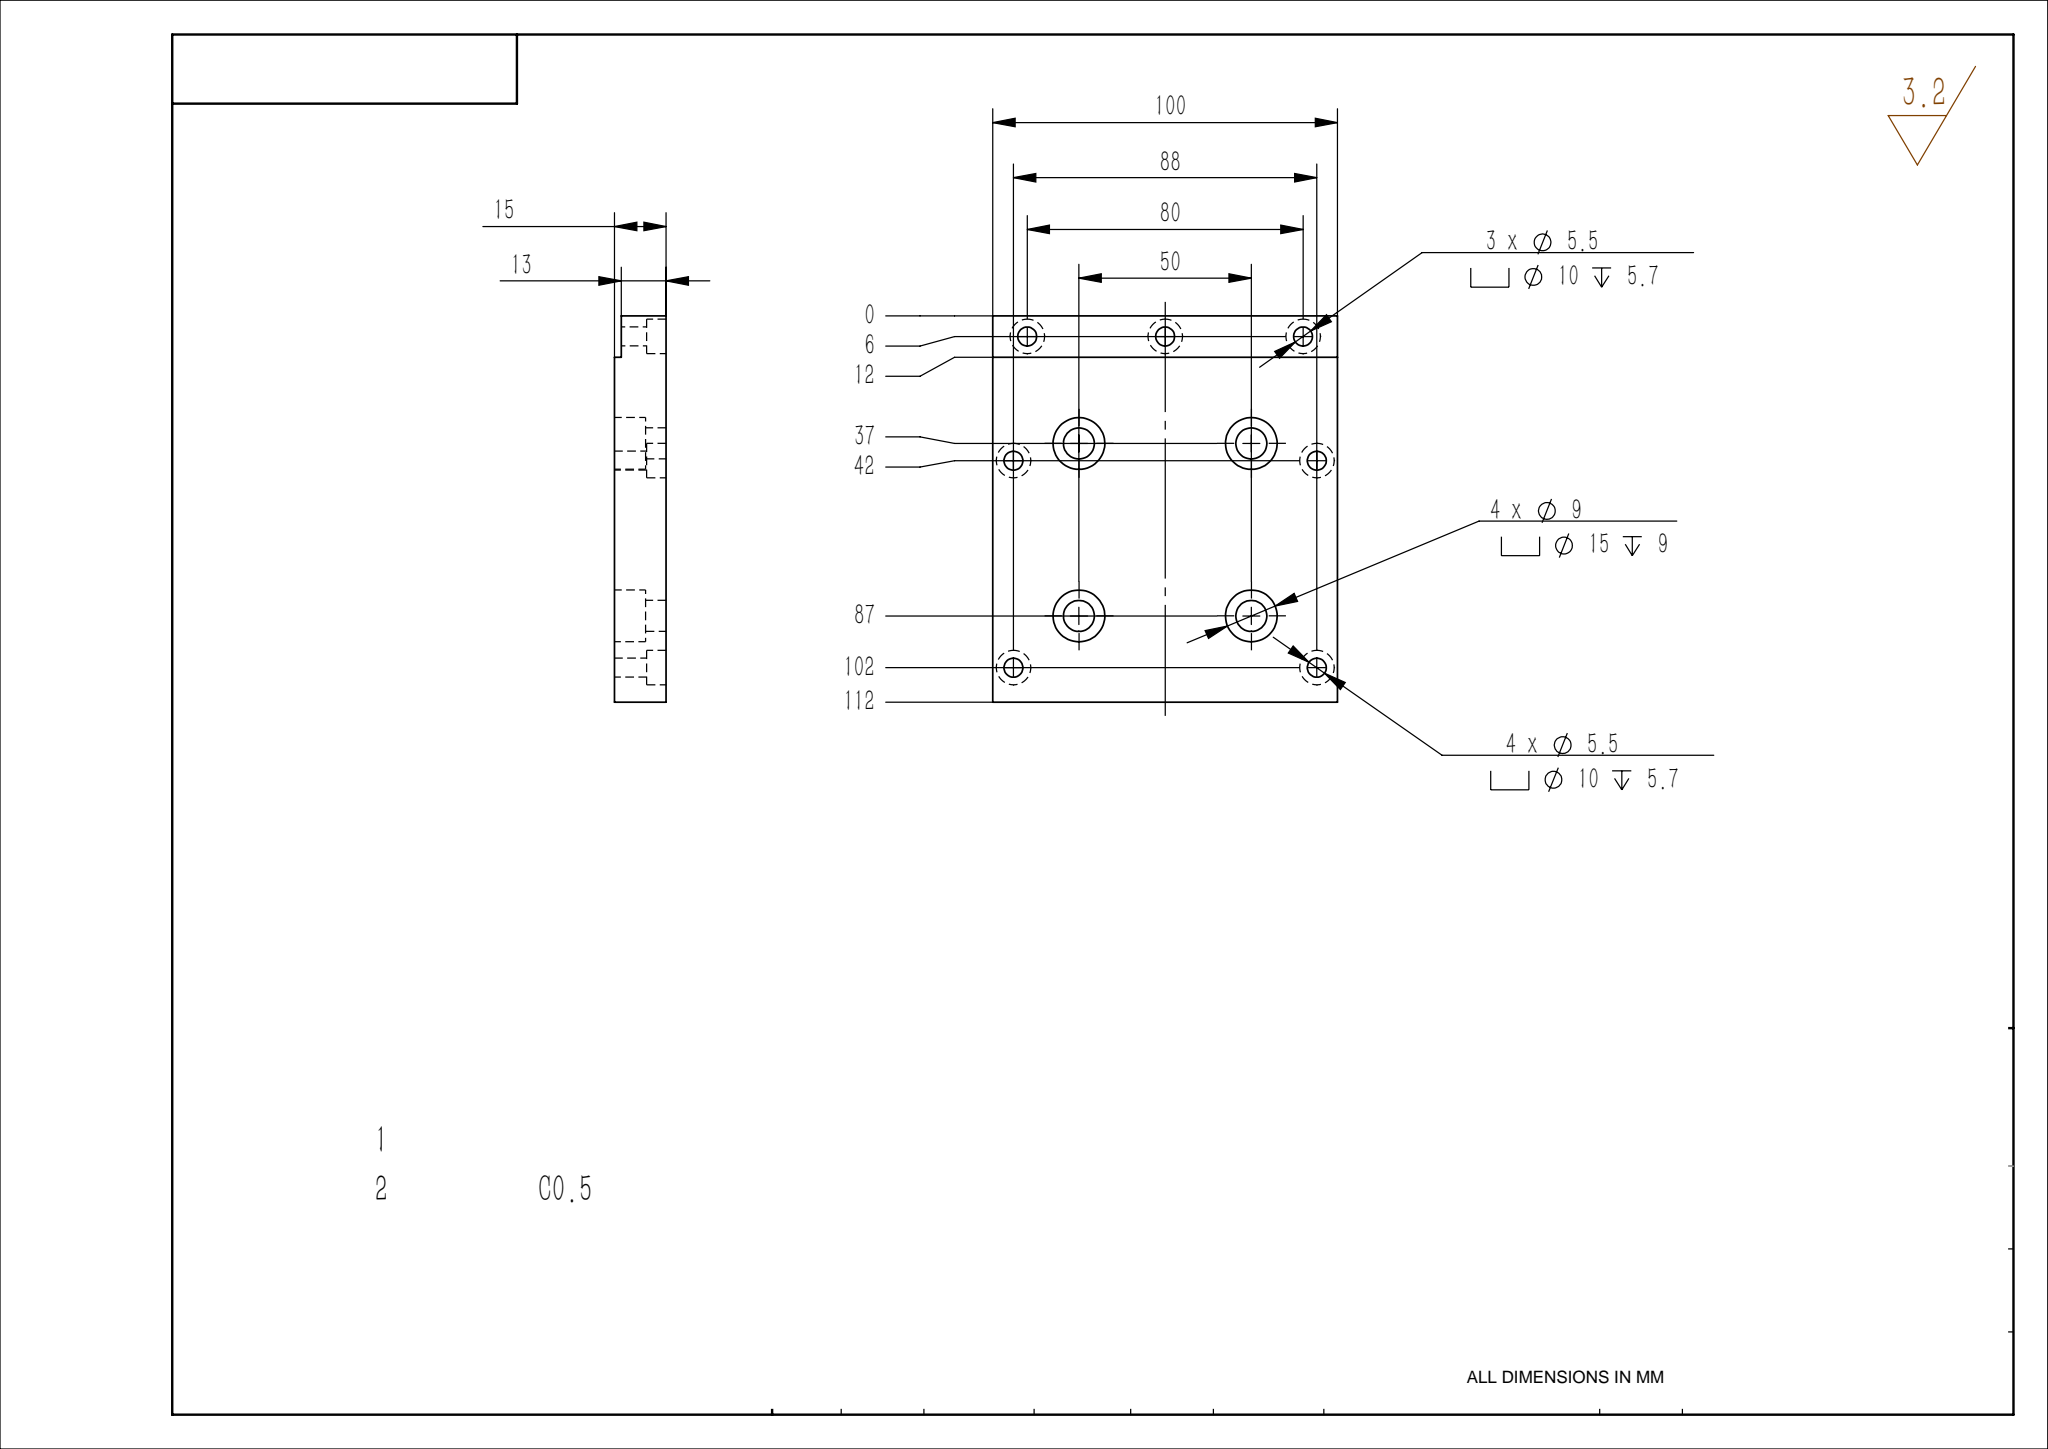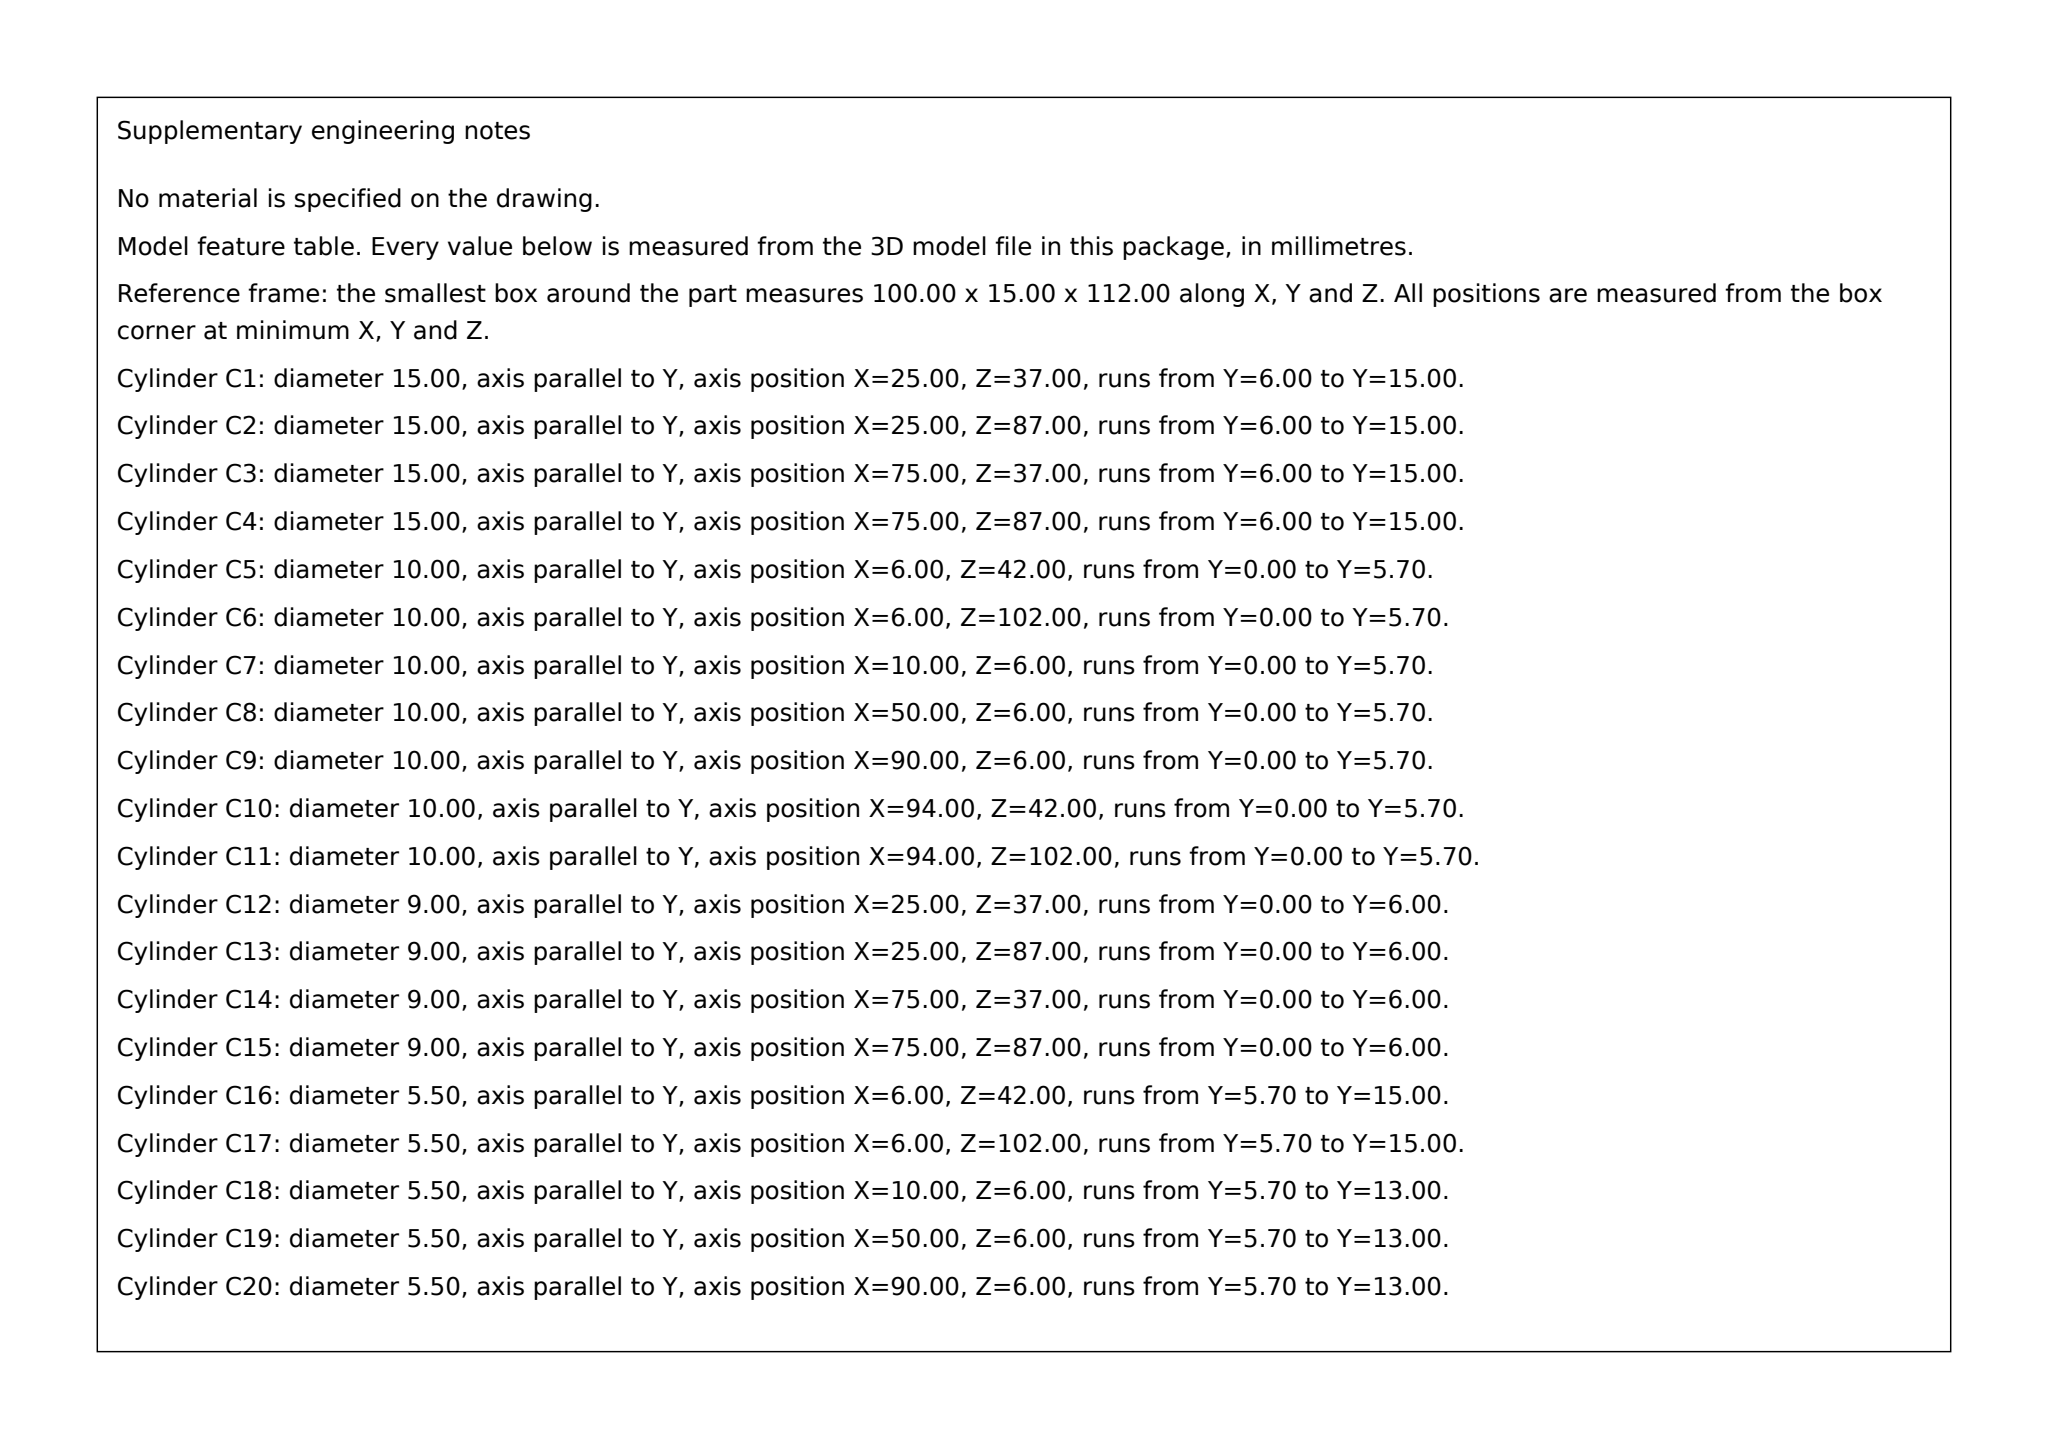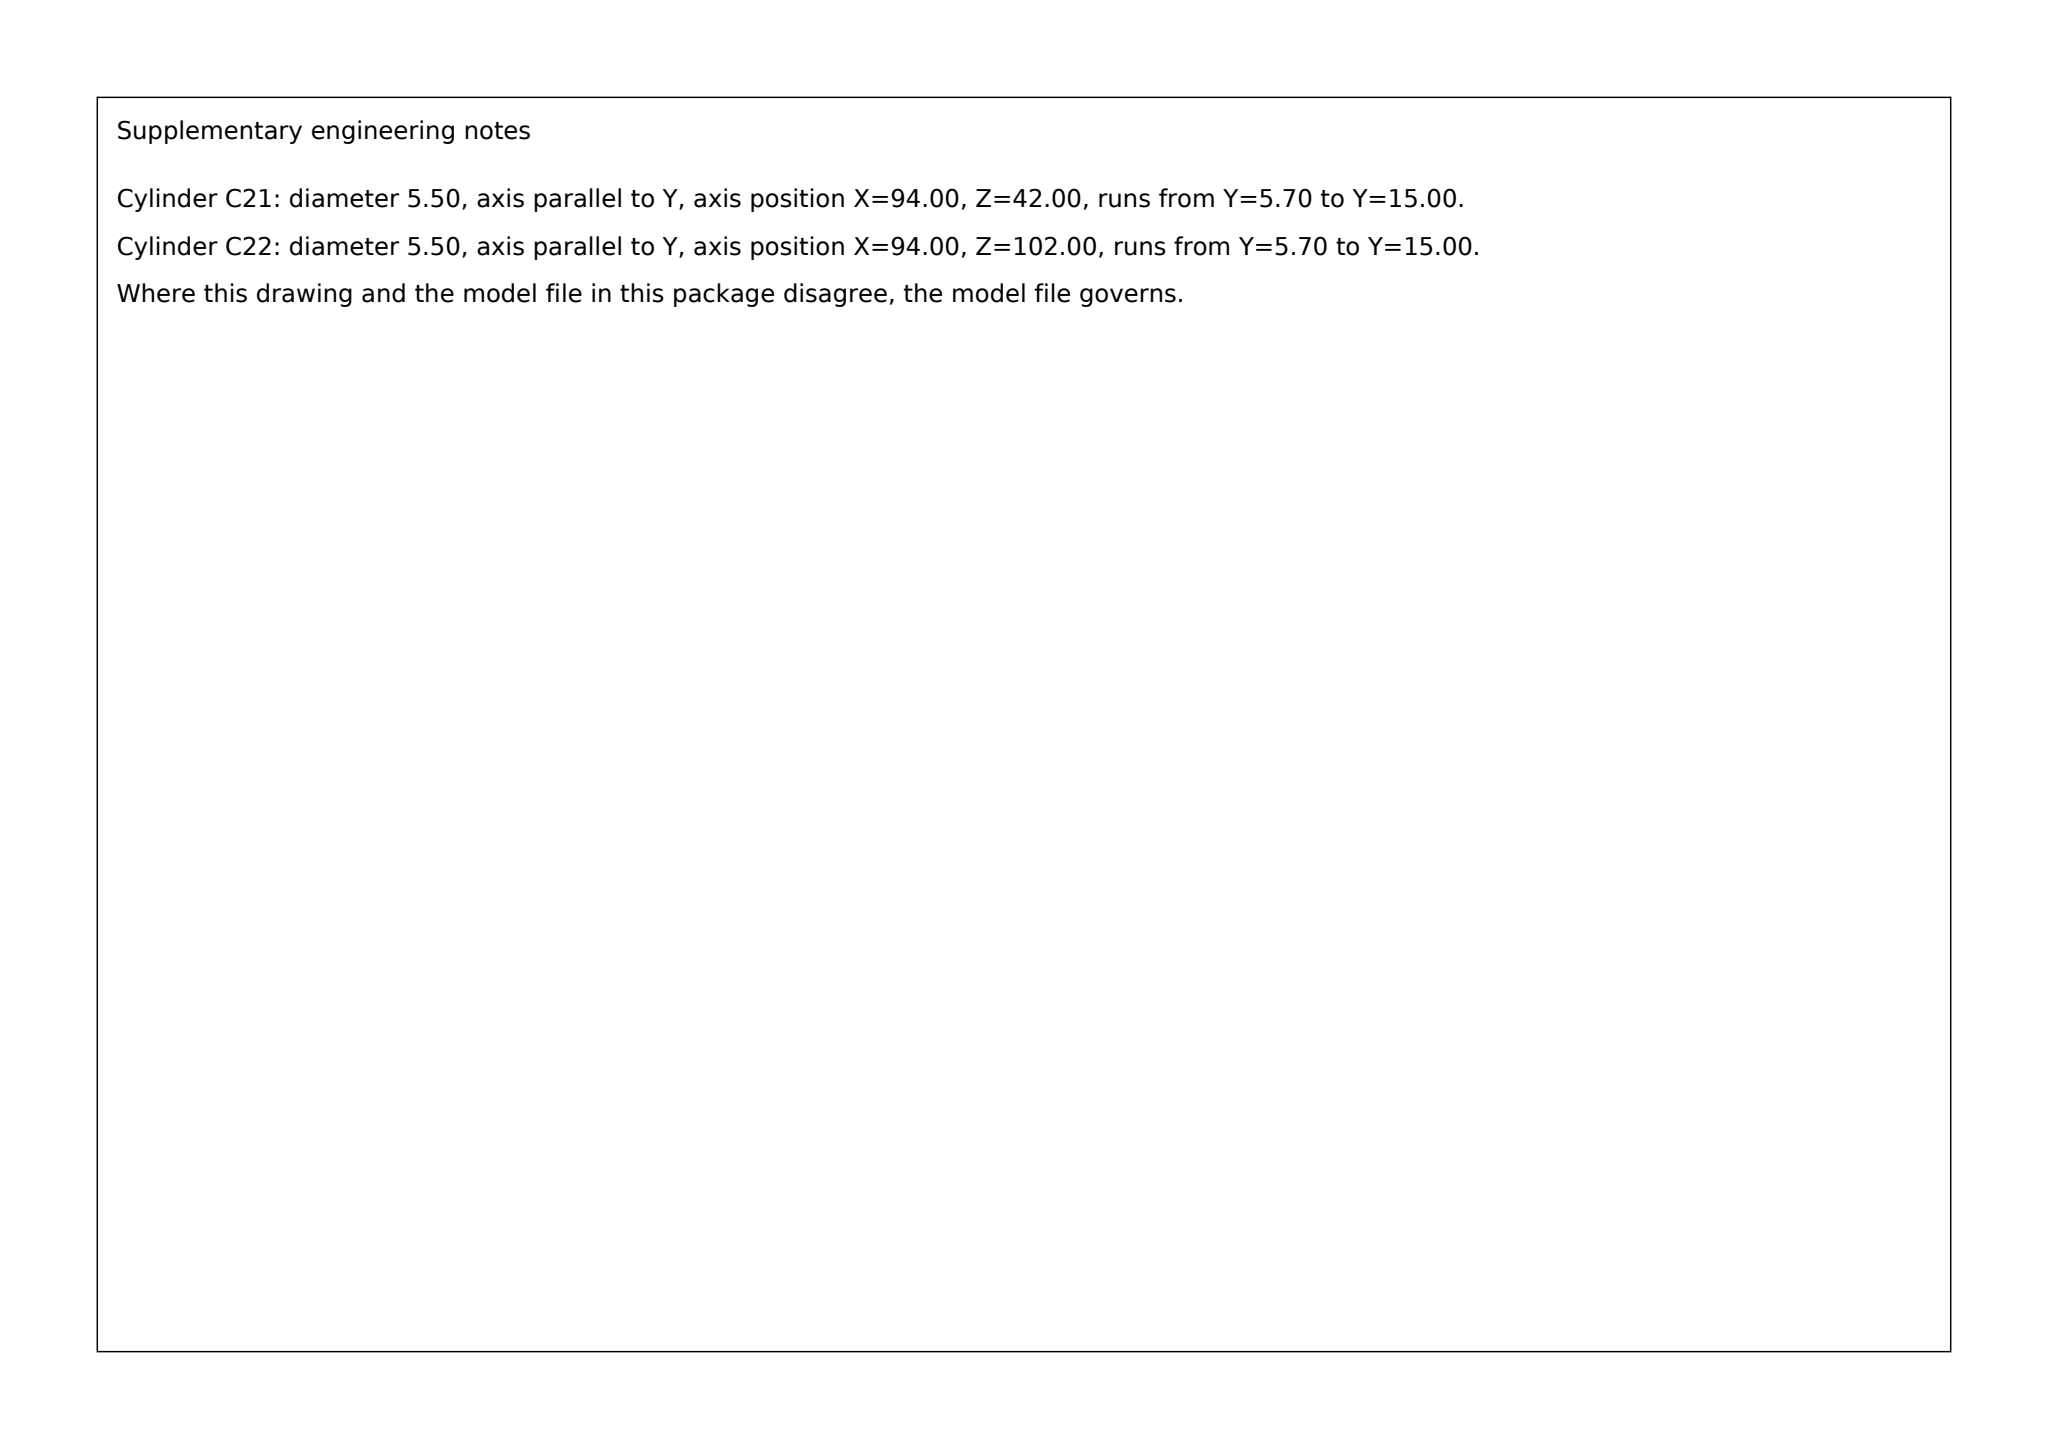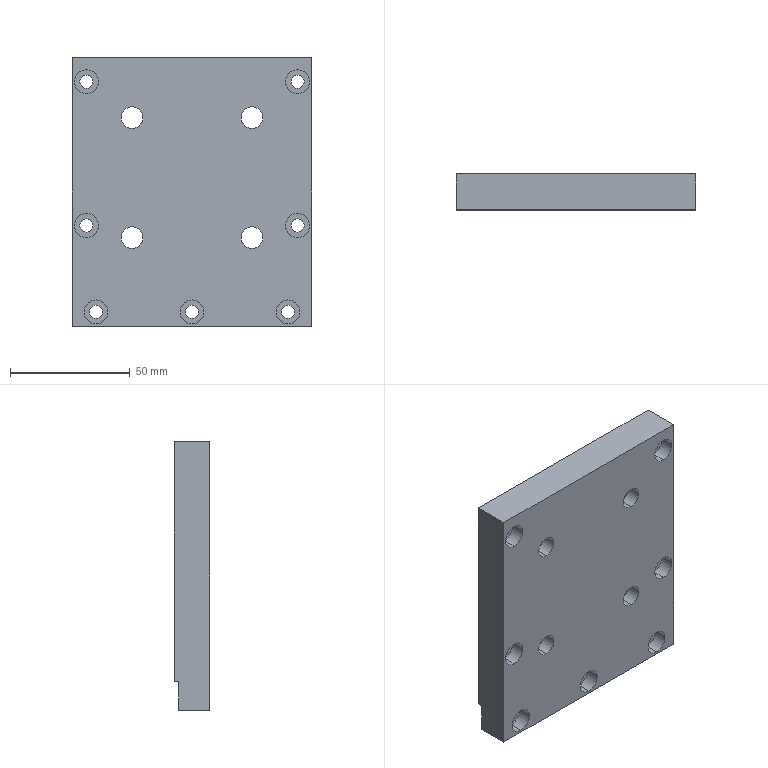Part | SolidWorks | mm | 1 solid | 63 faces | box 100 x 15 x 112 mm | volume 153174 mm3 | cylinder 44 | plane 19 | commonest cylinder face diameters 10 x14 5.5 x14 15 x8 9 x8
build123d program:
from build123d import *

# Parameters (mm, degrees)
SKETCH1_W                                         = 100
SKETCH1_H                                         = 112
BOSS_EXTRUDE1_DEPTH                               = 15
SKETCH2_W                                         = 100
SKETCH2_H                                         = 12
CUT_EXTRUDE1_DEPTH                                = 2
HOLE_SIZE_ACCORDING_TO_HEXAGON_SOCKET_D           = 9
HOLE_SIZE_ACCORDING_TO_HEXAGON_SOCKET_CBORE_D     = 15
HOLE_SIZE_ACCORDING_TO_HEXAGON_SOCKET_CBORE_DEPTH = 9
HOLE_SIZE_ACCORDING_TO_HEXAGON_SO_2_D             = 5.5
HOLE_SIZE_ACCORDING_TO_HEXAGON_SO_2_CBORE_D       = 10
HOLE_SIZE_ACCORDING_TO_HEXAGON_SO_2_CBORE_DEPTH   = 5.7
HOLE_SIZE_ACCORDING_TO_HEXAGON_SO_3_D             = 5.5
HOLE_SIZE_ACCORDING_TO_HEXAGON_SO_3_CBORE_D       = 10
HOLE_SIZE_ACCORDING_TO_HEXAGON_SO_3_CBORE_DEPTH   = 5.7


with BuildPart() as part:
    # Sketch1 → Boss-Extrude1 (new body)
    with BuildSketch(Plane(origin=(0, 0, 0), x_dir=(1, 0, 0), z_dir=(0, 1, 0))):
        Rectangle(SKETCH1_W, SKETCH1_H)
    extrude(amount=BOSS_EXTRUDE1_DEPTH)

    # Sketch2 → Cut-Extrude1 (cut)
    with BuildSketch(Plane(origin=(0, 15, 0), x_dir=(1, 0, 0), z_dir=(0, 1, 0))):
        with Locations((0, 50)):
            Rectangle(SKETCH2_W, SKETCH2_H)
    extrude(amount=-CUT_EXTRUDE1_DEPTH, mode=Mode.SUBTRACT)

    # Hole Size _ according to_ Hexagon Socket (through all)
    with Locations(Plane(origin=(0, 15, 0), x_dir=(1, 0, 0), z_dir=(0, 1, 0))):
        with Locations((-25, 19), (25, 19), (25, -31), (-25, -31)):
            CounterBoreHole(HOLE_SIZE_ACCORDING_TO_HEXAGON_SOCKET_D / 2, HOLE_SIZE_ACCORDING_TO_HEXAGON_SOCKET_CBORE_D / 2, HOLE_SIZE_ACCORDING_TO_HEXAGON_SOCKET_CBORE_DEPTH)

    # Hole Size _ according to_ Hexagon So 2 (through all)
    with Locations(Plane(origin=(0, 0, 0), x_dir=(-1, 0, 0), z_dir=(0, -1, 0))):
        with Locations((44, -46), (44, 14), (-44, -46), (-44, 14)):
            CounterBoreHole(HOLE_SIZE_ACCORDING_TO_HEXAGON_SO_2_D / 2, HOLE_SIZE_ACCORDING_TO_HEXAGON_SO_2_CBORE_D / 2, HOLE_SIZE_ACCORDING_TO_HEXAGON_SO_2_CBORE_DEPTH)

    # Hole Size _ according to_ Hexagon So 3 (through all)
    with Locations(Plane(origin=(0, 0, 0), x_dir=(-1, 0, 0), z_dir=(0, -1, 0))):
        with Locations((-40, 50), (0, 50), (40, 50)):
            CounterBoreHole(HOLE_SIZE_ACCORDING_TO_HEXAGON_SO_3_D / 2, HOLE_SIZE_ACCORDING_TO_HEXAGON_SO_3_CBORE_D / 2, HOLE_SIZE_ACCORDING_TO_HEXAGON_SO_3_CBORE_DEPTH)


solid = part.part